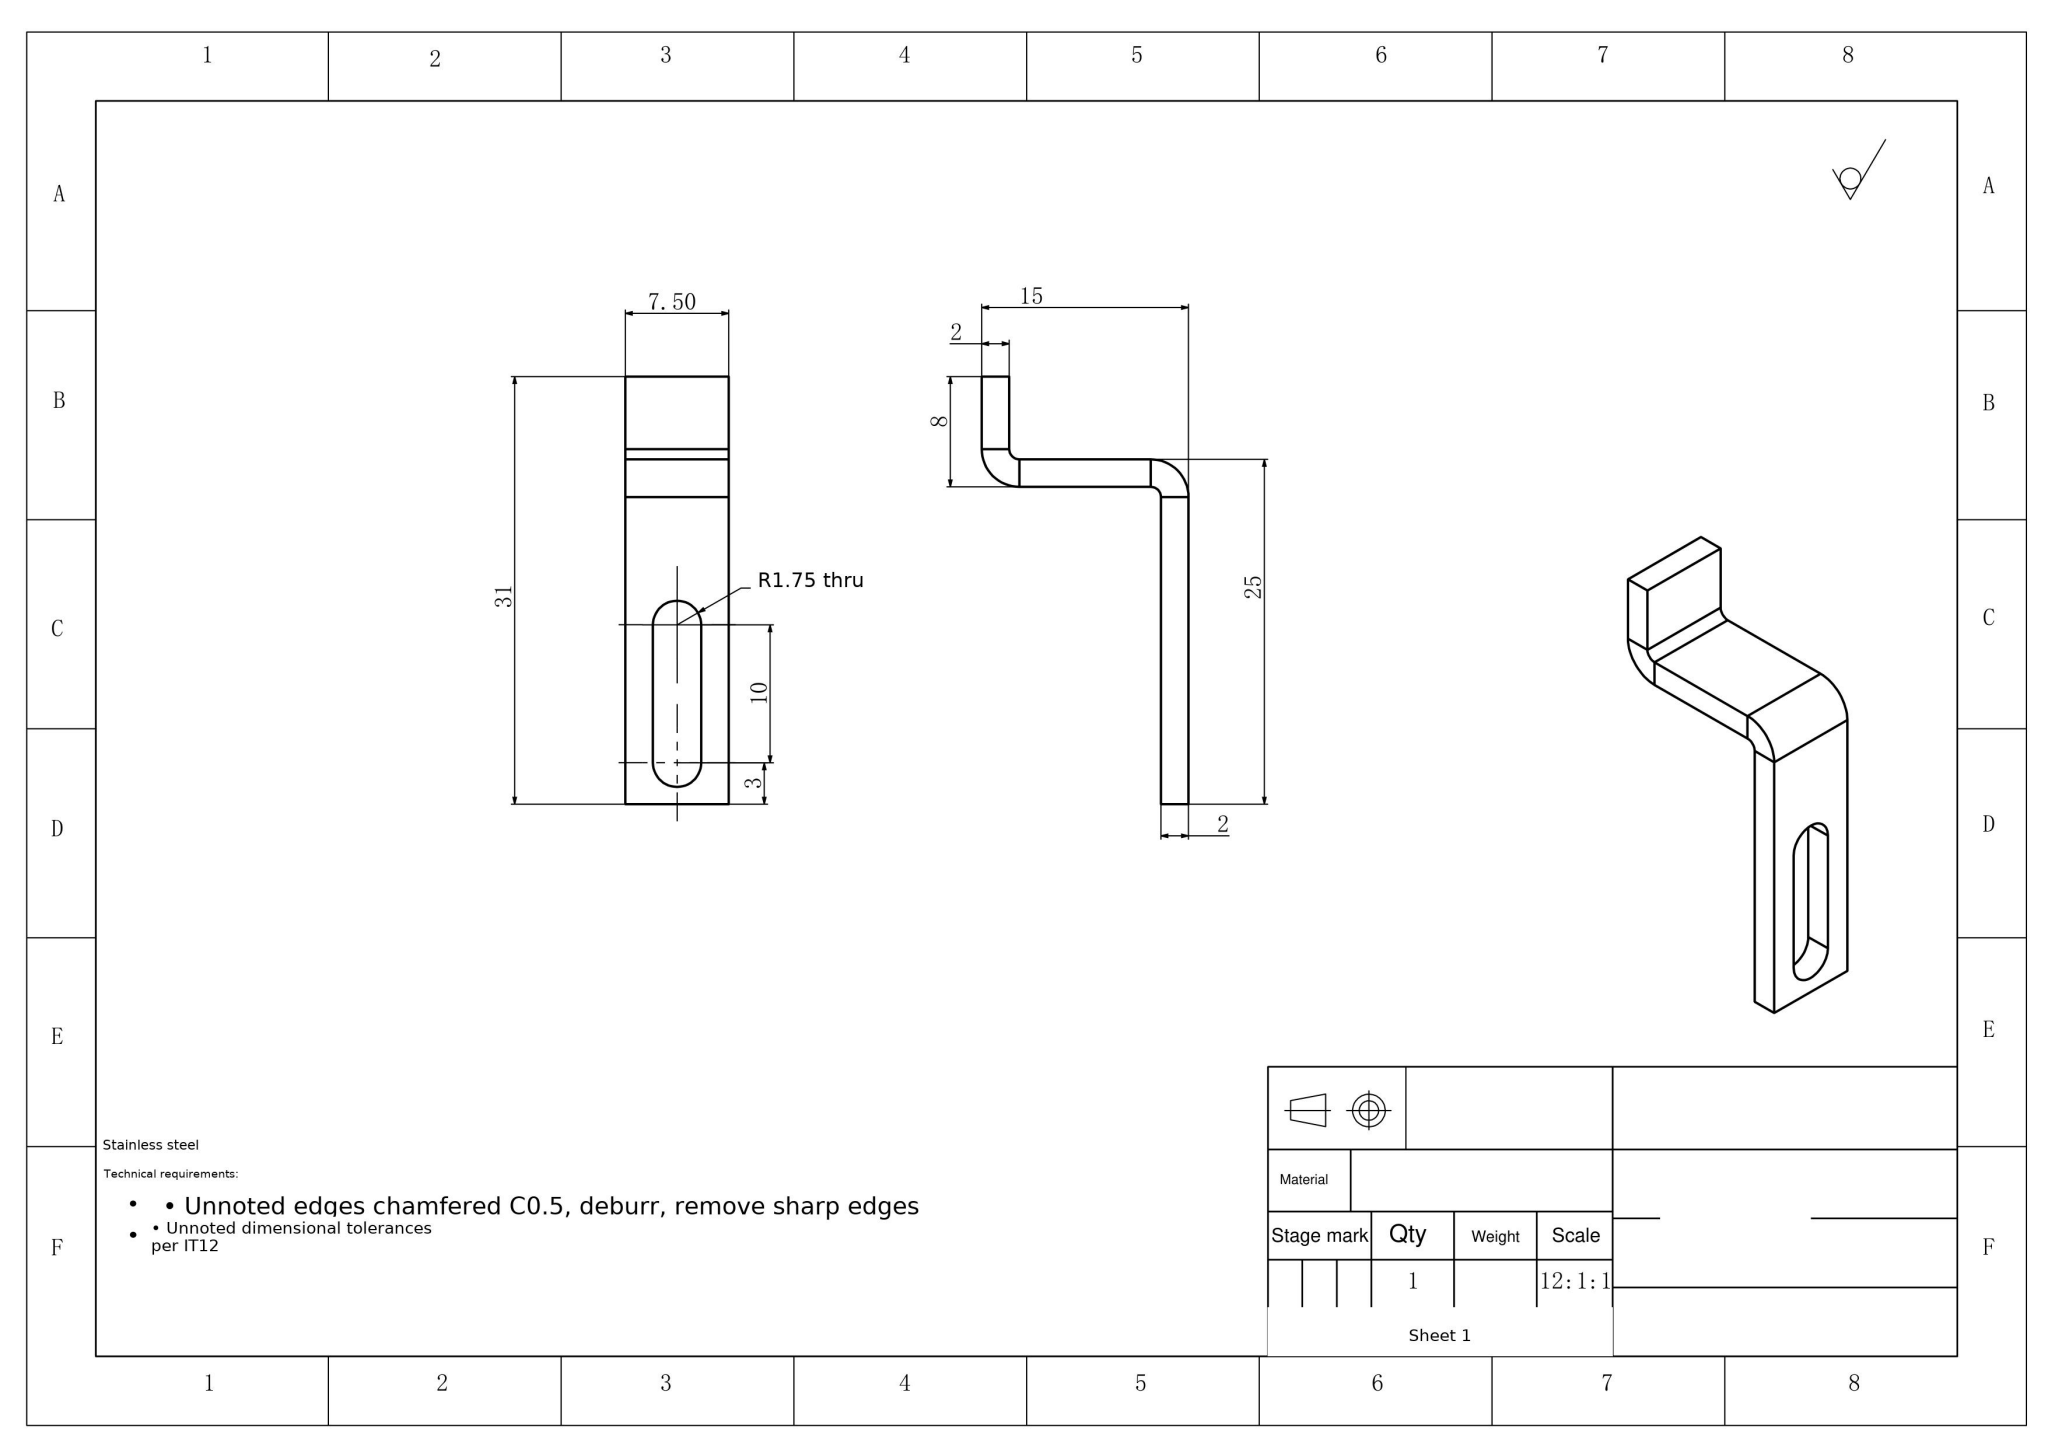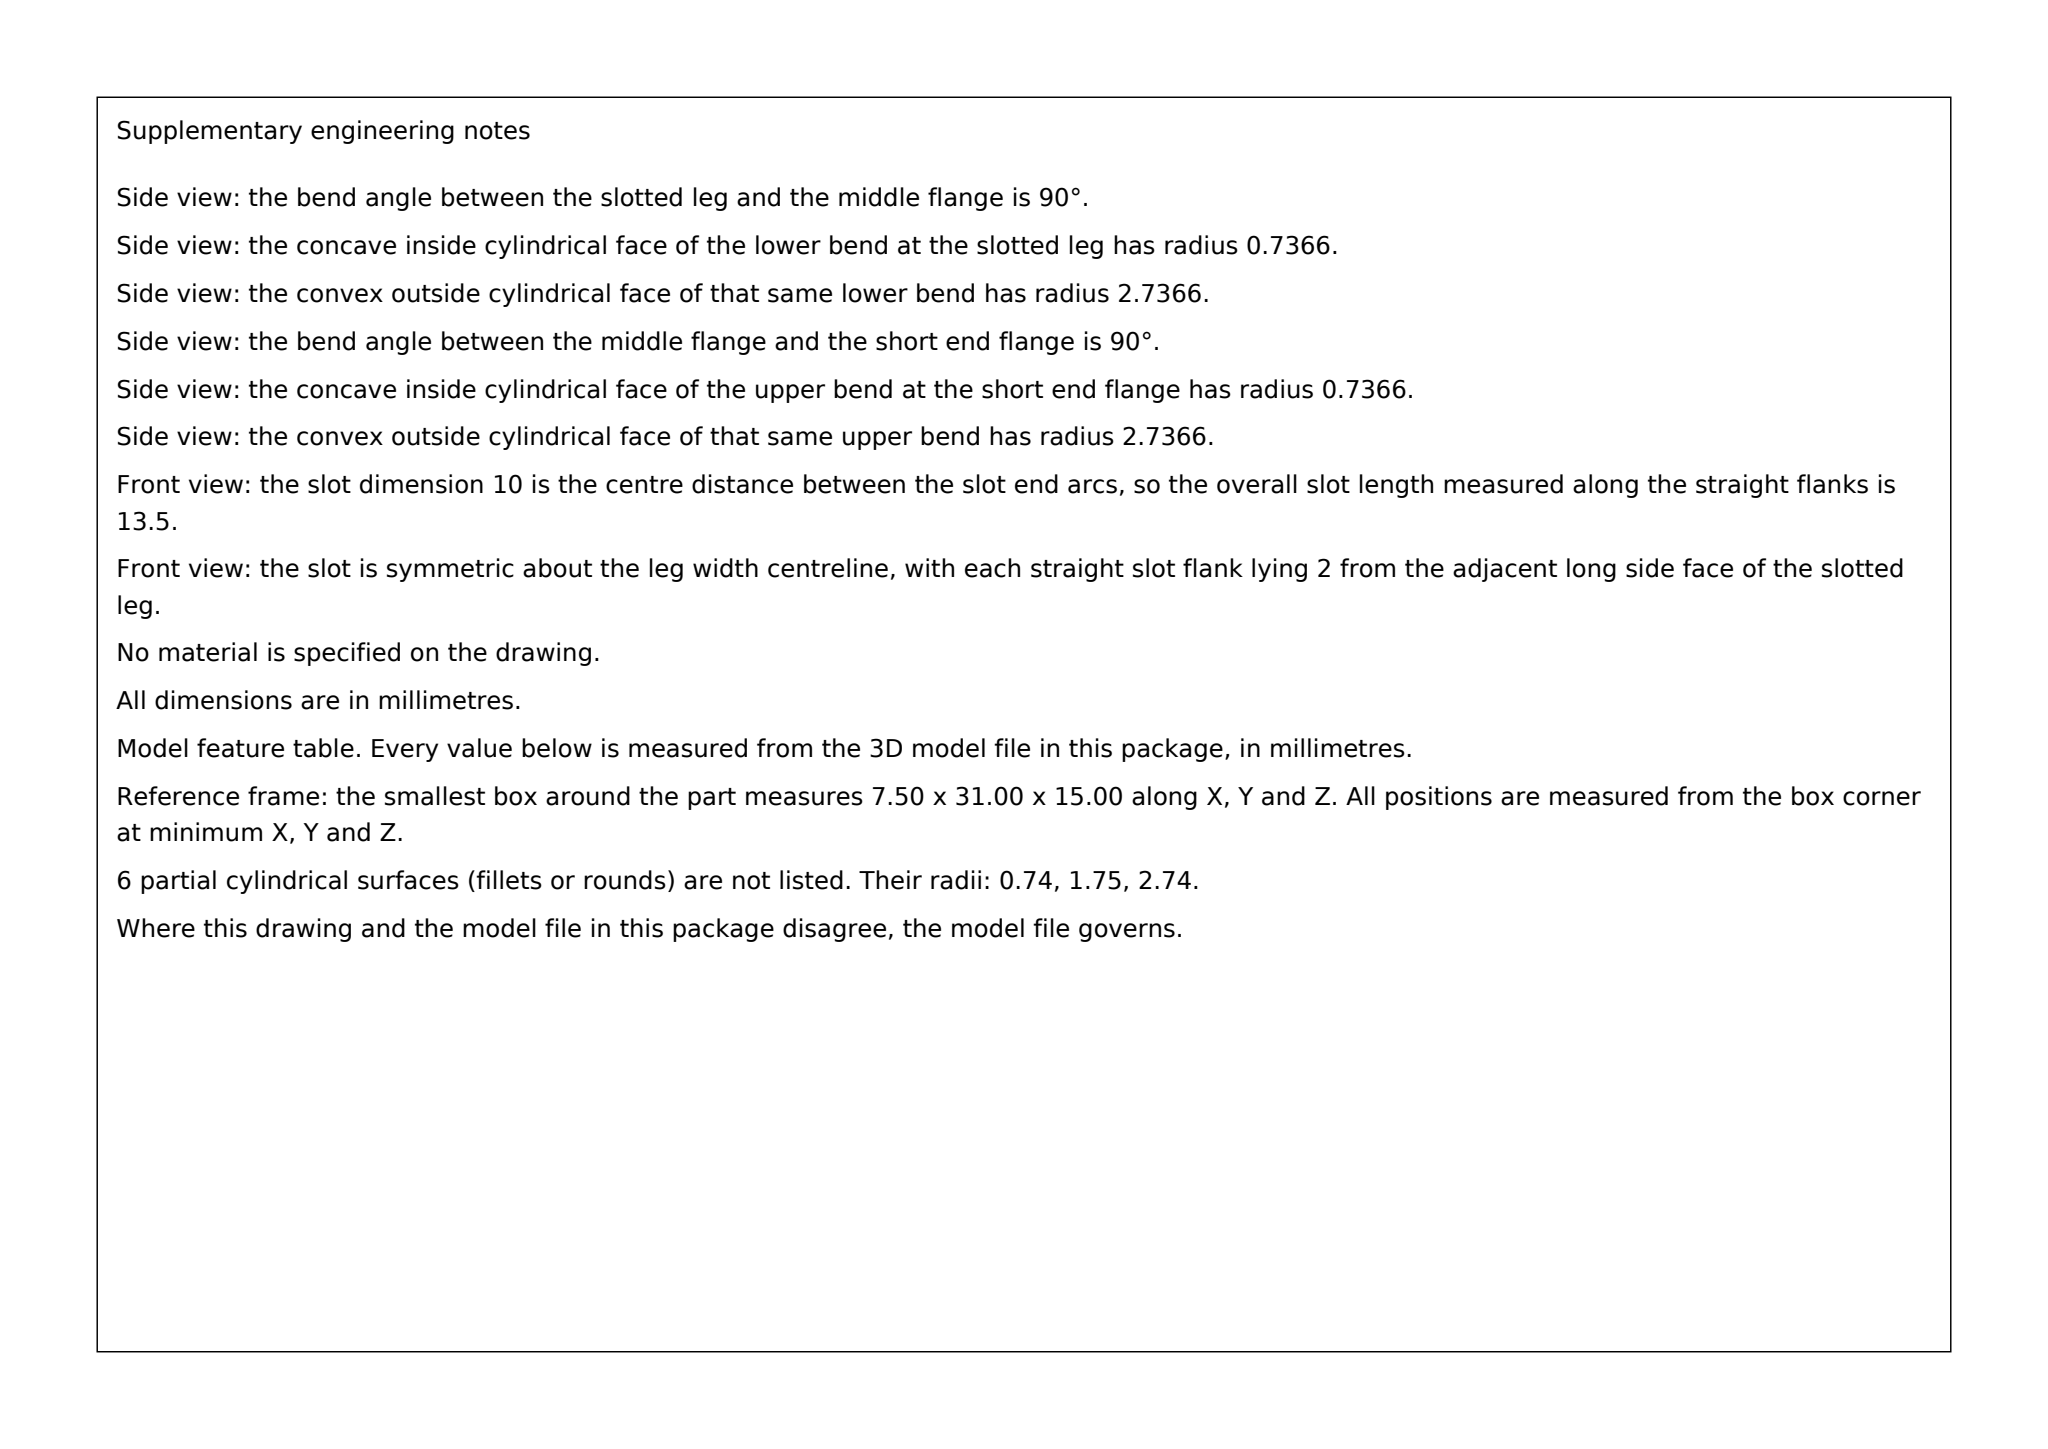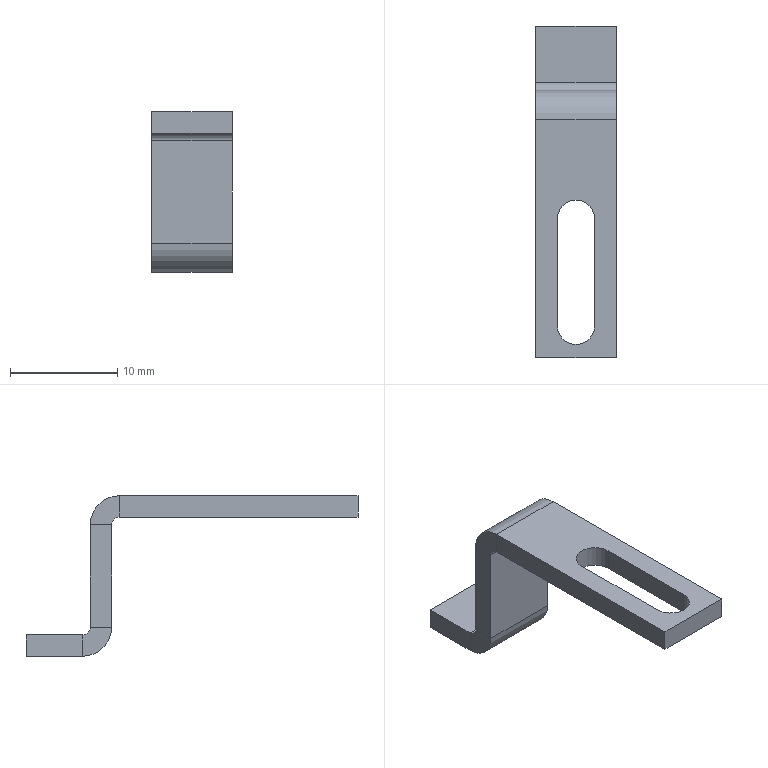Part | SolidWorks | mm | material Stainless steel | 1 solid | 26 faces | box 7.5 x 31 x 15 mm | volume 548 mm3 | plane 20 | cylinder 6 | commonest cylinder face diameters 3.5 x2 5.473 x2 1.473 x2
Drawing notes:
BEND FILLETS: 2X R0.74 INSIDE, 2X R2.74 OUTSIDE (DEL BALLOON 11) | from the solid: Cylinders dia 1.473 (R0.74) x2 and dia 5.473 (R2.74) x2, axis X, at y/z 22.26/12.26 and 25.74/2.74, length 7.5 = full width; inner/outer radii of the two 90 deg bends
STEP:
#1=CARTESIAN_POINT('',(3.75,12.5,-12.263));
#2=VERTEX_POINT('',#1);
#3=CARTESIAN_POINT('',(3.75,10.5,-12.263));
#4=VERTEX_POINT('',#3);
#5=CARTESIAN_POINT('',(3.75,12.5,-12.263));
#6=DIRECTION('',(0.,-1.,-0.));
#7=VECTOR('',#6,1000.);
#8=LINE('',#5,#7);
#9=EDGE_CURVE('',#2,#4,#8,.T.);
#10=ORIENTED_EDGE('',*,*,#9,.F.);
#11=CARTESIAN_POINT('',(3.75,12.5,-2.737));
#12=VERTEX_POINT('',#11);
#13=CARTESIAN_POINT('',(3.75,12.5,0.));
#14=DIRECTION('',(0.,0.,-1.));
#15=VECTOR('',#14,1000.);
#16=LINE('',#13,#15);
#17=EDGE_CURVE('',#12,#2,#16,.T.);
#18=ORIENTED_EDGE('',*,*,#17,.F.);
#19=CARTESIAN_POINT('',(3.75,10.5,-2.737));
#20=VERTEX_POINT('',#19);
#21=CARTESIAN_POINT('',(3.75,10.5,-2.737));
#22=DIRECTION('',(0.,1.,0.));
#23=VECTOR('',#22,1000.);
#24=LINE('',#21,#23);
#25=EDGE_CURVE('',#20,#12,#24,.T.);
#26=ORIENTED_EDGE('',*,*,#25,.F.);
#27=CARTESIAN_POINT('',(3.75,10.5,-15.));
#28=DIRECTION('',(0.,0.,-1.));
#29=VECTOR('',#28,1000.);
#30=LINE('',#27,#29);
#31=EDGE_CURVE('',#20,#4,#30,.T.);
#32=ORIENTED_EDGE('',*,*,#31,.T.);
#33=EDGE_LOOP('',(#10,#18,#26,#32));
#34=FACE_OUTER_BOUND('',#33,.T.);
#35=CARTESIAN_POINT('',(3.75,12.5,-15.));
#36=DIRECTION('',(-1.,0.,0.));
#37=DIRECTION('',(0.,0.,1.));
#38=AXIS2_PLACEMENT_3D('',#35,#36,#37);
#39=PLANE('',#38);
#40=ADVANCED_FACE('',(#34),#39,.F.);
#41=CARTESIAN_POINT('',(-3.75,12.5,-12.263));
#42=VERTEX_POINT('',#41);
#43=CARTESIAN_POINT('',(-3.75,10.5,-12.263));
#44=VERTEX_POINT('',#43);
#45=CARTESIAN_POINT('',(-3.75,12.5,-12.263));
#46=DIRECTION('',(-0.,-1.,-0.));
#47=VECTOR('',#46,1000.);
#48=LINE('',#45,#47);
#49=EDGE_CURVE('',#42,#44,#48,.T.);
#50=ORIENTED_EDGE('',*,*,#49,.T.);
#51=CARTESIAN_POINT('',(-3.75,10.5,-2.737));
#52=VERTEX_POINT('',#51);
#53=CARTESIAN_POINT('',(-3.75,10.5,-2.));
#54=DIRECTION('',(0.,-0.,1.));
#55=VECTOR('',#54,1000.);
#56=LINE('',#53,#55);
#57=EDGE_CURVE('',#44,#52,#56,.T.);
#58=ORIENTED_EDGE('',*,*,#57,.T.);
#59=CARTESIAN_POINT('',(-3.75,12.5,-2.737));
#60=VERTEX_POINT('',#59);
#61=CARTESIAN_POINT('',(-3.75,12.5,-2.737));
#62=DIRECTION('',(0.,1.,0.));
#63=VECTOR('',#62,1000.);
#64=LINE('',#61,#63);
#65=EDGE_CURVE('',#52,#60,#64,.T.);
#66=ORIENTED_EDGE('',*,*,#65,.T.);
#67=CARTESIAN_POINT('',(-3.75,12.5,0.));
#68=DIRECTION('',(0.,-0.,1.));
#69=VECTOR('',#68,1000.);
#70=LINE('',#67,#69);
#71=EDGE_CURVE('',#42,#60,#70,.T.);
#72=ORIENTED_EDGE('',*,*,#71,.F.);
#73=EDGE_LOOP('',(#50,#58,#66,#72));
#74=FACE_OUTER_BOUND('',#73,.T.);
#75=CARTESIAN_POINT('',(-3.75,12.5,-2.));
#76=DIRECTION('',(1.,0.,0.));
#77=DIRECTION('',(0.,0.,-1.));
#78=AXIS2_PLACEMENT_3D('',#75,#76,#77);
#79=PLANE('',#78);
#80=ADVANCED_FACE('',(#74),#79,.F.);
#81=CARTESIAN_POINT('',(-3.75,12.5,-12.263));
#82=DIRECTION('',(1.,0.,-0.));
#83=VECTOR('',#82,1000.);
#84=LINE('',#81,#83);
#85=EDGE_CURVE('',#42,#2,#84,.T.);
#86=ORIENTED_EDGE('',*,*,#85,.F.);
#87=ORIENTED_EDGE('',*,*,#71,.T.);
#88=CARTESIAN_POINT('',(-3.75,12.5,-2.737));
#89=DIRECTION('',(-1.,0.,0.));
#90=VECTOR('',#89,1000.);
#91=LINE('',#88,#90);
#92=EDGE_CURVE('',#12,#60,#91,.T.);
#93=ORIENTED_EDGE('',*,*,#92,.F.);
#94=ORIENTED_EDGE('',*,*,#17,.T.);
#95=EDGE_LOOP('',(#86,#87,#93,#94));
#96=FACE_OUTER_BOUND('',#95,.T.);
#97=CARTESIAN_POINT('',(0.,12.5,0.));
#98=DIRECTION('',(0.,-1.,-0.));
#99=DIRECTION('',(0.,0.,-1.));
#100=AXIS2_PLACEMENT_3D('',#97,#98,#99);
#101=PLANE('',#100);
#102=ADVANCED_FACE('',(#96),#101,.F.);
#103=ORIENTED_EDGE('',*,*,#57,.F.);
#104=CARTESIAN_POINT('',(-3.75,10.5,-12.263));
#105=DIRECTION('',(1.,0.,-0.));
#106=VECTOR('',#105,1000.);
#107=LINE('',#104,#106);
#108=EDGE_CURVE('',#44,#4,#107,.T.);
#109=ORIENTED_EDGE('',*,*,#108,.T.);
#110=ORIENTED_EDGE('',*,*,#31,.F.);
#111=CARTESIAN_POINT('',(-3.75,10.5,-2.737));
#112=DIRECTION('',(1.,0.,0.));
#113=VECTOR('',#112,1000.);
#114=LINE('',#111,#113);
#115=EDGE_CURVE('',#52,#20,#114,.T.);
#116=ORIENTED_EDGE('',*,*,#115,.F.);
#117=EDGE_LOOP('',(#103,#109,#110,#116));
#118=FACE_OUTER_BOUND('',#117,.T.);
#119=CARTESIAN_POINT('',(0.,10.5,0.));
#120=DIRECTION('',(0.,-1.,-0.));
#121=DIRECTION('',(0.,0.,-1.));
#122=AXIS2_PLACEMENT_3D('',#119,#120,#121);
#123=PLANE('',#122);
#124=ADVANCED_FACE('',(#118),#123,.T.);
#125=CARTESIAN_POINT('',(3.75,-12.5,-2.));
#126=VERTEX_POINT('',#125);
#127=CARTESIAN_POINT('',(3.75,9.763,-2.));
#128=VERTEX_POINT('',#127);
#129=CARTESIAN_POINT('',(3.75,-12.5,-2.));
#130=DIRECTION('',(0.,1.,0.));
#131=VECTOR('',#130,1000.);
#132=LINE('',#129,#131);
#133=EDGE_CURVE('',#126,#128,#132,.T.);
#134=ORIENTED_EDGE('',*,*,#133,.T.);
#135=CARTESIAN_POINT('',(3.75,9.763,0.));
#136=VERTEX_POINT('',#135);
#137=CARTESIAN_POINT('',(3.75,9.763,-2.));
#138=DIRECTION('',(0.,0.,1.));
#139=VECTOR('',#138,1000.);
#140=LINE('',#137,#139);
#141=EDGE_CURVE('',#128,#136,#140,.T.);
#142=ORIENTED_EDGE('',*,*,#141,.T.);
#143=CARTESIAN_POINT('',(3.75,-12.5,0.));
#144=VERTEX_POINT('',#143);
#145=CARTESIAN_POINT('',(3.75,-12.5,0.));
#146=DIRECTION('',(0.,1.,0.));
#147=VECTOR('',#146,1000.);
#148=LINE('',#145,#147);
#149=EDGE_CURVE('',#144,#136,#148,.T.);
#150=ORIENTED_EDGE('',*,*,#149,.F.);
#151=CARTESIAN_POINT('',(3.75,-12.5,-2.));
#152=DIRECTION('',(0.,0.,1.));
#153=VECTOR('',#152,1000.);
#154=LINE('',#151,#153);
#155=EDGE_CURVE('',#126,#144,#154,.T.);
#156=ORIENTED_EDGE('',*,*,#155,.F.);
#157=EDGE_LOOP('',(#134,#142,#150,#156));
#158=FACE_OUTER_BOUND('',#157,.T.);
#159=CARTESIAN_POINT('',(3.75,-12.5,-2.));
#160=DIRECTION('',(1.,0.,0.));
#161=DIRECTION('',(0.,0.,-1.));
#162=AXIS2_PLACEMENT_3D('',#159,#160,#161);
#163=PLANE('',#162);
#164=ADVANCED_FACE('',(#158),#163,.T.);
#165=CARTESIAN_POINT('',(1.75,0.5,-2.));
#166=VERTEX_POINT('',#165);
#167=CARTESIAN_POINT('',(-1.75,0.5,-2.));
#168=VERTEX_POINT('',#167);
#169=CARTESIAN_POINT('',(0.,0.5,-2.));
#170=DIRECTION('',(0.,0.,1.));
#171=DIRECTION('',(1.,0.,0.));
#172=AXIS2_PLACEMENT_3D('',#169,#170,#171);
#173=CIRCLE('',#172,1.75);
#174=EDGE_CURVE('',#166,#168,#173,.T.);
#175=ORIENTED_EDGE('',*,*,#174,.T.);
#176=CARTESIAN_POINT('',(-1.75,-9.5,-2.));
#177=VERTEX_POINT('',#176);
#178=CARTESIAN_POINT('',(-1.75,0.5,-2.));
#179=DIRECTION('',(0.,-1.,0.));
#180=VECTOR('',#179,1000.);
#181=LINE('',#178,#180);
#182=EDGE_CURVE('',#168,#177,#181,.T.);
#183=ORIENTED_EDGE('',*,*,#182,.T.);
#184=CARTESIAN_POINT('',(1.75,-9.5,-2.));
#185=VERTEX_POINT('',#184);
#186=CARTESIAN_POINT('',(0.,-9.5,-2.));
#187=DIRECTION('',(0.,0.,1.));
#188=DIRECTION('',(1.,0.,0.));
#189=AXIS2_PLACEMENT_3D('',#186,#187,#188);
#190=CIRCLE('',#189,1.75);
#191=EDGE_CURVE('',#177,#185,#190,.T.);
#192=ORIENTED_EDGE('',*,*,#191,.T.);
#193=CARTESIAN_POINT('',(1.75,0.5,-2.));
#194=DIRECTION('',(-0.,1.,0.));
#195=VECTOR('',#194,1000.);
#196=LINE('',#193,#195);
#197=EDGE_CURVE('',#185,#166,#196,.T.);
#198=ORIENTED_EDGE('',*,*,#197,.T.);
#199=EDGE_LOOP('',(#175,#183,#192,#198));
#200=FACE_BOUND('',#199,.T.);
#201=CARTESIAN_POINT('',(-3.75,9.763,-2.));
#202=VERTEX_POINT('',#201);
#203=CARTESIAN_POINT('',(-3.75,-12.5,-2.));
#204=VERTEX_POINT('',#203);
#205=CARTESIAN_POINT('',(-3.75,-12.5,-2.));
#206=DIRECTION('',(0.,-1.,0.));
#207=VECTOR('',#206,1000.);
#208=LINE('',#205,#207);
#209=EDGE_CURVE('',#202,#204,#208,.T.);
#210=ORIENTED_EDGE('',*,*,#209,.F.);
#211=CARTESIAN_POINT('',(3.75,9.763,-2.));
#212=DIRECTION('',(-1.,0.,0.));
#213=VECTOR('',#212,1000.);
#214=LINE('',#211,#213);
#215=EDGE_CURVE('',#128,#202,#214,.T.);
#216=ORIENTED_EDGE('',*,*,#215,.F.);
#217=ORIENTED_EDGE('',*,*,#133,.F.);
#218=CARTESIAN_POINT('',(-3.75,-12.5,-2.));
#219=DIRECTION('',(1.,0.,0.));
#220=VECTOR('',#219,1000.);
#221=LINE('',#218,#220);
#222=EDGE_CURVE('',#204,#126,#221,.T.);
#223=ORIENTED_EDGE('',*,*,#222,.F.);
#224=EDGE_LOOP('',(#210,#216,#217,#223));
#225=FACE_OUTER_BOUND('',#224,.T.);
#226=CARTESIAN_POINT('',(0.,0.,-2.));
#227=DIRECTION('',(0.,0.,-1.));
#228=DIRECTION('',(-1.,0.,0.));
#229=AXIS2_PLACEMENT_3D('',#226,#227,#228);
#230=PLANE('',#229);
#231=ADVANCED_FACE('',(#200,#225),#230,.T.);
#232=CARTESIAN_POINT('',(-1.75,0.5,0.));
#233=VERTEX_POINT('',#232);
#234=CARTESIAN_POINT('',(-1.75,-9.5,0.));
#235=VERTEX_POINT('',#234);
#236=CARTESIAN_POINT('',(-1.75,0.5,0.));
#237=DIRECTION('',(0.,-1.,0.));
#238=VECTOR('',#237,1000.);
#239=LINE('',#236,#238);
#240=EDGE_CURVE('',#233,#235,#239,.T.);
#241=ORIENTED_EDGE('',*,*,#240,.F.);
#242=CARTESIAN_POINT('',(1.75,0.5,0.));
#243=VERTEX_POINT('',#242);
#244=CARTESIAN_POINT('',(0.,0.5,0.));
#245=DIRECTION('',(0.,0.,1.));
#246=DIRECTION('',(1.,0.,0.));
#247=AXIS2_PLACEMENT_3D('',#244,#245,#246);
#248=CIRCLE('',#247,1.75);
#249=EDGE_CURVE('',#243,#233,#248,.T.);
#250=ORIENTED_EDGE('',*,*,#249,.F.);
#251=CARTESIAN_POINT('',(1.75,-9.5,0.));
#252=VERTEX_POINT('',#251);
#253=CARTESIAN_POINT('',(1.75,0.5,0.));
#254=DIRECTION('',(-0.,1.,0.));
#255=VECTOR('',#254,1000.);
#256=LINE('',#253,#255);
#257=EDGE_CURVE('',#252,#243,#256,.T.);
#258=ORIENTED_EDGE('',*,*,#257,.F.);
#259=CARTESIAN_POINT('',(0.,-9.5,0.));
#260=DIRECTION('',(0.,0.,1.));
#261=DIRECTION('',(1.,0.,0.));
#262=AXIS2_PLACEMENT_3D('',#259,#260,#261);
#263=CIRCLE('',#262,1.75);
#264=EDGE_CURVE('',#235,#252,#263,.T.);
#265=ORIENTED_EDGE('',*,*,#264,.F.);
#266=EDGE_LOOP('',(#241,#250,#258,#265));
#267=FACE_BOUND('',#266,.T.);
#268=CARTESIAN_POINT('',(-3.75,9.763,0.));
#269=VERTEX_POINT('',#268);
#270=CARTESIAN_POINT('',(3.75,9.763,0.));
#271=DIRECTION('',(-1.,0.,0.));
#272=VECTOR('',#271,1000.);
#273=LINE('',#270,#272);
#274=EDGE_CURVE('',#136,#269,#273,.T.);
#275=ORIENTED_EDGE('',*,*,#274,.T.);
#276=CARTESIAN_POINT('',(-3.75,-12.5,0.));
#277=VERTEX_POINT('',#276);
#278=CARTESIAN_POINT('',(-3.75,-12.5,0.));
#279=DIRECTION('',(0.,-1.,0.));
#280=VECTOR('',#279,1000.);
#281=LINE('',#278,#280);
#282=EDGE_CURVE('',#269,#277,#281,.T.);
#283=ORIENTED_EDGE('',*,*,#282,.T.);
#284=CARTESIAN_POINT('',(-3.75,-12.5,0.));
#285=DIRECTION('',(1.,0.,0.));
#286=VECTOR('',#285,1000.);
#287=LINE('',#284,#286);
#288=EDGE_CURVE('',#277,#144,#287,.T.);
#289=ORIENTED_EDGE('',*,*,#288,.T.);
#290=ORIENTED_EDGE('',*,*,#149,.T.);
#291=EDGE_LOOP('',(#275,#283,#289,#290));
#292=FACE_OUTER_BOUND('',#291,.T.);
#293=CARTESIAN_POINT('',(0.,0.,0.));
#294=DIRECTION('',(0.,0.,-1.));
#295=DIRECTION('',(-1.,0.,0.));
#296=AXIS2_PLACEMENT_3D('',#293,#294,#295);
#297=PLANE('',#296);
#298=ADVANCED_FACE('',(#267,#292),#297,.F.);
#299=ORIENTED_EDGE('',*,*,#288,.F.);
#300=CARTESIAN_POINT('',(-3.75,-12.5,-2.));
#301=DIRECTION('',(0.,0.,1.));
#302=VECTOR('',#301,1000.);
#303=LINE('',#300,#302);
#304=EDGE_CURVE('',#204,#277,#303,.T.);
#305=ORIENTED_EDGE('',*,*,#304,.F.);
#306=ORIENTED_EDGE('',*,*,#222,.T.);
#307=ORIENTED_EDGE('',*,*,#155,.T.);
#308=EDGE_LOOP('',(#299,#305,#306,#307));
#309=FACE_OUTER_BOUND('',#308,.T.);
#310=CARTESIAN_POINT('',(-3.75,-12.5,-2.));
#311=DIRECTION('',(0.,-1.,0.));
#312=DIRECTION('',(0.,0.,-1.));
#313=AXIS2_PLACEMENT_3D('',#310,#311,#312);
#314=PLANE('',#313);
#315=ADVANCED_FACE('',(#309),#314,.T.);
#316=CARTESIAN_POINT('',(-3.75,9.763,-2.));
#317=DIRECTION('',(0.,0.,1.));
#318=VECTOR('',#317,1000.);
#319=LINE('',#316,#318);
#320=EDGE_CURVE('',#202,#269,#319,.T.);
#321=ORIENTED_EDGE('',*,*,#320,.F.);
#322=ORIENTED_EDGE('',*,*,#209,.T.);
#323=ORIENTED_EDGE('',*,*,#304,.T.);
#324=ORIENTED_EDGE('',*,*,#282,.F.);
#325=EDGE_LOOP('',(#321,#322,#323,#324));
#326=FACE_OUTER_BOUND('',#325,.T.);
#327=CARTESIAN_POINT('',(-3.75,-12.5,-2.));
#328=DIRECTION('',(-1.,0.,0.));
#329=DIRECTION('',(0.,0.,1.));
#330=AXIS2_PLACEMENT_3D('',#327,#328,#329);
#331=PLANE('',#330);
#332=ADVANCED_FACE('',(#326),#331,.T.);
#333=ORIENTED_EDGE('',*,*,#249,.T.);
#334=CARTESIAN_POINT('',(-1.75,0.5,-2.));
#335=DIRECTION('',(0.,0.,1.));
#336=VECTOR('',#335,1000.);
#337=LINE('',#334,#336);
#338=EDGE_CURVE('',#168,#233,#337,.T.);
#339=ORIENTED_EDGE('',*,*,#338,.F.);
#340=ORIENTED_EDGE('',*,*,#174,.F.);
#341=CARTESIAN_POINT('',(1.75,0.5,-2.));
#342=DIRECTION('',(0.,0.,1.));
#343=VECTOR('',#342,1000.);
#344=LINE('',#341,#343);
#345=EDGE_CURVE('',#166,#243,#344,.T.);
#346=ORIENTED_EDGE('',*,*,#345,.T.);
#347=EDGE_LOOP('',(#333,#339,#340,#346));
#348=FACE_OUTER_BOUND('',#347,.T.);
#349=CARTESIAN_POINT('',(0.,0.5,-2.));
#350=DIRECTION('',(0.,0.,1.));
#351=DIRECTION('',(1.,0.,0.));
#352=AXIS2_PLACEMENT_3D('',#349,#350,#351);
#353=CYLINDRICAL_SURFACE('',#352,1.75);
#354=ADVANCED_FACE('',(#348),#353,.F.);
#355=ORIENTED_EDGE('',*,*,#257,.T.);
#356=ORIENTED_EDGE('',*,*,#345,.F.);
#357=ORIENTED_EDGE('',*,*,#197,.F.);
#358=CARTESIAN_POINT('',(1.75,-9.5,-2.));
#359=DIRECTION('',(0.,0.,1.));
#360=VECTOR('',#359,1000.);
#361=LINE('',#358,#360);
#362=EDGE_CURVE('',#185,#252,#361,.T.);
#363=ORIENTED_EDGE('',*,*,#362,.T.);
#364=EDGE_LOOP('',(#355,#356,#357,#363));
#365=FACE_OUTER_BOUND('',#364,.T.);
#366=CARTESIAN_POINT('',(1.75,0.5,-2.));
#367=DIRECTION('',(1.,0.,0.));
#368=DIRECTION('',(-0.,1.,0.));
#369=AXIS2_PLACEMENT_3D('',#366,#367,#368);
#370=PLANE('',#369);
#371=ADVANCED_FACE('',(#365),#370,.F.);
#372=ORIENTED_EDGE('',*,*,#264,.T.);
#373=ORIENTED_EDGE('',*,*,#362,.F.);
#374=ORIENTED_EDGE('',*,*,#191,.F.);
#375=CARTESIAN_POINT('',(-1.75,-9.5,-2.));
#376=DIRECTION('',(0.,0.,1.));
#377=VECTOR('',#376,1000.);
#378=LINE('',#375,#377);
#379=EDGE_CURVE('',#177,#235,#378,.T.);
#380=ORIENTED_EDGE('',*,*,#379,.T.);
#381=EDGE_LOOP('',(#372,#373,#374,#380));
#382=FACE_OUTER_BOUND('',#381,.T.);
#383=CARTESIAN_POINT('',(0.,-9.5,-2.));
#384=DIRECTION('',(0.,0.,1.));
#385=DIRECTION('',(1.,0.,0.));
#386=AXIS2_PLACEMENT_3D('',#383,#384,#385);
#387=CYLINDRICAL_SURFACE('',#386,1.75);
#388=ADVANCED_FACE('',(#382),#387,.F.);
#389=ORIENTED_EDGE('',*,*,#240,.T.);
#390=ORIENTED_EDGE('',*,*,#379,.F.);
#391=ORIENTED_EDGE('',*,*,#182,.F.);
#392=ORIENTED_EDGE('',*,*,#338,.T.);
#393=EDGE_LOOP('',(#389,#390,#391,#392));
#394=FACE_OUTER_BOUND('',#393,.T.);
#395=CARTESIAN_POINT('',(-1.75,0.5,-2.));
#396=DIRECTION('',(-1.,-0.,0.));
#397=DIRECTION('',(0.,-1.,0.));
#398=AXIS2_PLACEMENT_3D('',#395,#396,#397);
#399=PLANE('',#398);
#400=ADVANCED_FACE('',(#394),#399,.F.);
#401=ORIENTED_EDGE('',*,*,#65,.F.);
#402=CARTESIAN_POINT('',(-3.75,9.763,-2.737));
#403=DIRECTION('',(-1.,0.,0.));
#404=DIRECTION('',(0.,0.,-1.));
#405=AXIS2_PLACEMENT_3D('',#402,#403,#404);
#406=CIRCLE('',#405,0.7366);
#407=EDGE_CURVE('',#202,#52,#406,.T.);
#408=ORIENTED_EDGE('',*,*,#407,.F.);
#409=ORIENTED_EDGE('',*,*,#320,.T.);
#410=CARTESIAN_POINT('',(-3.75,9.763,-2.737));
#411=DIRECTION('',(-1.,0.,0.));
#412=DIRECTION('',(0.,0.,-1.));
#413=AXIS2_PLACEMENT_3D('',#410,#411,#412);
#414=CIRCLE('',#413,2.737);
#415=EDGE_CURVE('',#269,#60,#414,.T.);
#416=ORIENTED_EDGE('',*,*,#415,.T.);
#417=EDGE_LOOP('',(#401,#408,#409,#416));
#418=FACE_OUTER_BOUND('',#417,.T.);
#419=CARTESIAN_POINT('',(-3.75,9.763,-2.737));
#420=DIRECTION('',(-1.,0.,0.));
#421=DIRECTION('',(0.,0.,1.));
#422=AXIS2_PLACEMENT_3D('',#419,#420,#421);
#423=PLANE('',#422);
#424=ADVANCED_FACE('',(#418),#423,.T.);
#425=CARTESIAN_POINT('',(3.75,9.763,-2.737));
#426=DIRECTION('',(1.,0.,0.));
#427=DIRECTION('',(0.,0.,-1.));
#428=AXIS2_PLACEMENT_3D('',#425,#426,#427);
#429=CIRCLE('',#428,0.7366);
#430=EDGE_CURVE('',#20,#128,#429,.T.);
#431=ORIENTED_EDGE('',*,*,#430,.F.);
#432=ORIENTED_EDGE('',*,*,#25,.T.);
#433=CARTESIAN_POINT('',(3.75,9.763,-2.737));
#434=DIRECTION('',(1.,0.,0.));
#435=DIRECTION('',(0.,0.,-1.));
#436=AXIS2_PLACEMENT_3D('',#433,#434,#435);
#437=CIRCLE('',#436,2.737);
#438=EDGE_CURVE('',#12,#136,#437,.T.);
#439=ORIENTED_EDGE('',*,*,#438,.T.);
#440=ORIENTED_EDGE('',*,*,#141,.F.);
#441=EDGE_LOOP('',(#431,#432,#439,#440));
#442=FACE_OUTER_BOUND('',#441,.T.);
#443=CARTESIAN_POINT('',(3.75,9.763,-2.737));
#444=DIRECTION('',(-1.,0.,0.));
#445=DIRECTION('',(0.,0.,1.));
#446=AXIS2_PLACEMENT_3D('',#443,#444,#445);
#447=PLANE('',#446);
#448=ADVANCED_FACE('',(#442),#447,.F.);
#449=ORIENTED_EDGE('',*,*,#274,.F.);
#450=ORIENTED_EDGE('',*,*,#438,.F.);
#451=ORIENTED_EDGE('',*,*,#92,.T.);
#452=ORIENTED_EDGE('',*,*,#415,.F.);
#453=EDGE_LOOP('',(#449,#450,#451,#452));
#454=FACE_OUTER_BOUND('',#453,.T.);
#455=CARTESIAN_POINT('',(3.75,9.763,-2.737));
#456=DIRECTION('',(1.,0.,0.));
#457=DIRECTION('',(0.,1.,0.));
#458=AXIS2_PLACEMENT_3D('',#455,#456,#457);
#459=CYLINDRICAL_SURFACE('',#458,2.737);
#460=ADVANCED_FACE('',(#454),#459,.T.);
#461=ORIENTED_EDGE('',*,*,#215,.T.);
#462=ORIENTED_EDGE('',*,*,#407,.T.);
#463=ORIENTED_EDGE('',*,*,#115,.T.);
#464=ORIENTED_EDGE('',*,*,#430,.T.);
#465=EDGE_LOOP('',(#461,#462,#463,#464));
#466=FACE_OUTER_BOUND('',#465,.T.);
#467=CARTESIAN_POINT('',(3.75,9.763,-2.737));
#468=DIRECTION('',(1.,0.,0.));
#469=DIRECTION('',(0.,1.,0.));
#470=AXIS2_PLACEMENT_3D('',#467,#468,#469);
#471=CYLINDRICAL_SURFACE('',#470,0.7366);
#472=ADVANCED_FACE('',(#466),#471,.F.);
#473=CARTESIAN_POINT('',(3.75,13.237,-13.));
#474=VERTEX_POINT('',#473);
#475=CARTESIAN_POINT('',(3.75,13.237,-15.));
#476=VERTEX_POINT('',#475);
#477=CARTESIAN_POINT('',(3.75,13.237,-15.));
#478=DIRECTION('',(0.,0.,-1.));
#479=VECTOR('',#478,1000.);
#480=LINE('',#477,#479);
#481=EDGE_CURVE('',#474,#476,#480,.T.);
#482=ORIENTED_EDGE('',*,*,#481,.F.);
#483=CARTESIAN_POINT('',(3.75,13.237,-12.263));
#484=DIRECTION('',(1.,0.,-0.));
#485=DIRECTION('',(0.,0.,1.));
#486=AXIS2_PLACEMENT_3D('',#483,#484,#485);
#487=CIRCLE('',#486,0.7366);
#488=EDGE_CURVE('',#2,#474,#487,.T.);
#489=ORIENTED_EDGE('',*,*,#488,.F.);
#490=ORIENTED_EDGE('',*,*,#9,.T.);
#491=CARTESIAN_POINT('',(3.75,13.237,-12.263));
#492=DIRECTION('',(1.,0.,-0.));
#493=DIRECTION('',(0.,0.,1.));
#494=AXIS2_PLACEMENT_3D('',#491,#492,#493);
#495=CIRCLE('',#494,2.737);
#496=EDGE_CURVE('',#4,#476,#495,.T.);
#497=ORIENTED_EDGE('',*,*,#496,.T.);
#498=EDGE_LOOP('',(#482,#489,#490,#497));
#499=FACE_OUTER_BOUND('',#498,.T.);
#500=CARTESIAN_POINT('',(3.75,13.237,-12.263));
#501=DIRECTION('',(1.,0.,-0.));
#502=DIRECTION('',(-0.,0.,-1.));
#503=AXIS2_PLACEMENT_3D('',#500,#501,#502);
#504=PLANE('',#503);
#505=ADVANCED_FACE('',(#499),#504,.T.);
#506=CARTESIAN_POINT('',(-3.75,13.237,-13.));
#507=VERTEX_POINT('',#506);
#508=CARTESIAN_POINT('',(-3.75,13.237,-12.263));
#509=DIRECTION('',(-1.,0.,0.));
#510=DIRECTION('',(0.,0.,1.));
#511=AXIS2_PLACEMENT_3D('',#508,#509,#510);
#512=CIRCLE('',#511,0.7366);
#513=EDGE_CURVE('',#507,#42,#512,.T.);
#514=ORIENTED_EDGE('',*,*,#513,.F.);
#515=CARTESIAN_POINT('',(-3.75,13.237,-15.));
#516=VERTEX_POINT('',#515);
#517=CARTESIAN_POINT('',(-3.75,13.237,-13.));
#518=DIRECTION('',(0.,0.,-1.));
#519=VECTOR('',#518,1000.);
#520=LINE('',#517,#519);
#521=EDGE_CURVE('',#507,#516,#520,.T.);
#522=ORIENTED_EDGE('',*,*,#521,.T.);
#523=CARTESIAN_POINT('',(-3.75,13.237,-12.263));
#524=DIRECTION('',(-1.,0.,0.));
#525=DIRECTION('',(0.,0.,1.));
#526=AXIS2_PLACEMENT_3D('',#523,#524,#525);
#527=CIRCLE('',#526,2.737);
#528=EDGE_CURVE('',#516,#44,#527,.T.);
#529=ORIENTED_EDGE('',*,*,#528,.T.);
#530=ORIENTED_EDGE('',*,*,#49,.F.);
#531=EDGE_LOOP('',(#514,#522,#529,#530));
#532=FACE_OUTER_BOUND('',#531,.T.);
#533=CARTESIAN_POINT('',(-3.75,13.237,-12.263));
#534=DIRECTION('',(1.,0.,-0.));
#535=DIRECTION('',(-0.,0.,-1.));
#536=AXIS2_PLACEMENT_3D('',#533,#534,#535);
#537=PLANE('',#536);
#538=ADVANCED_FACE('',(#532),#537,.F.);
#539=ORIENTED_EDGE('',*,*,#108,.F.);
#540=ORIENTED_EDGE('',*,*,#528,.F.);
#541=CARTESIAN_POINT('',(3.75,13.237,-15.));
#542=DIRECTION('',(1.,0.,0.));
#543=VECTOR('',#542,1000.);
#544=LINE('',#541,#543);
#545=EDGE_CURVE('',#516,#476,#544,.T.);
#546=ORIENTED_EDGE('',*,*,#545,.T.);
#547=ORIENTED_EDGE('',*,*,#496,.F.);
#548=EDGE_LOOP('',(#539,#540,#546,#547));
#549=FACE_OUTER_BOUND('',#548,.T.);
#550=CARTESIAN_POINT('',(-3.75,13.237,-12.263));
#551=DIRECTION('',(-1.,0.,0.));
#552=DIRECTION('',(-0.,0.,-1.));
#553=AXIS2_PLACEMENT_3D('',#550,#551,#552);
#554=CYLINDRICAL_SURFACE('',#553,2.737);
#555=ADVANCED_FACE('',(#549),#554,.T.);
#556=ORIENTED_EDGE('',*,*,#85,.T.);
#557=ORIENTED_EDGE('',*,*,#488,.T.);
#558=CARTESIAN_POINT('',(3.75,13.237,-13.));
#559=DIRECTION('',(-1.,0.,0.));
#560=VECTOR('',#559,1000.);
#561=LINE('',#558,#560);
#562=EDGE_CURVE('',#474,#507,#561,.T.);
#563=ORIENTED_EDGE('',*,*,#562,.T.);
#564=ORIENTED_EDGE('',*,*,#513,.T.);
#565=EDGE_LOOP('',(#556,#557,#563,#564));
#566=FACE_OUTER_BOUND('',#565,.T.);
#567=CARTESIAN_POINT('',(-3.75,13.237,-12.263));
#568=DIRECTION('',(-1.,0.,0.));
#569=DIRECTION('',(-0.,0.,-1.));
#570=AXIS2_PLACEMENT_3D('',#567,#568,#569);
#571=CYLINDRICAL_SURFACE('',#570,0.7366);
#572=ADVANCED_FACE('',(#566),#571,.F.);
#573=ORIENTED_EDGE('',*,*,#481,.T.);
#574=CARTESIAN_POINT('',(3.75,18.5,-15.));
#575=VERTEX_POINT('',#574);
#576=CARTESIAN_POINT('',(3.75,-0.,-15.));
#577=DIRECTION('',(0.,-1.,0.));
#578=VECTOR('',#577,1000.);
#579=LINE('',#576,#578);
#580=EDGE_CURVE('',#575,#476,#579,.T.);
#581=ORIENTED_EDGE('',*,*,#580,.F.);
#582=CARTESIAN_POINT('',(3.75,18.5,-13.));
#583=VERTEX_POINT('',#582);
#584=CARTESIAN_POINT('',(3.75,18.5,-15.));
#585=DIRECTION('',(0.,0.,1.));
#586=VECTOR('',#585,1000.);
#587=LINE('',#584,#586);
#588=EDGE_CURVE('',#575,#583,#587,.T.);
#589=ORIENTED_EDGE('',*,*,#588,.T.);
#590=CARTESIAN_POINT('',(3.75,12.5,-13.));
#591=DIRECTION('',(0.,-1.,0.));
#592=VECTOR('',#591,1000.);
#593=LINE('',#590,#592);
#594=EDGE_CURVE('',#583,#474,#593,.T.);
#595=ORIENTED_EDGE('',*,*,#594,.T.);
#596=EDGE_LOOP('',(#573,#581,#589,#595));
#597=FACE_OUTER_BOUND('',#596,.T.);
#598=CARTESIAN_POINT('',(3.75,12.5,-15.));
#599=DIRECTION('',(-1.,0.,0.));
#600=DIRECTION('',(0.,0.,1.));
#601=AXIS2_PLACEMENT_3D('',#598,#599,#600);
#602=PLANE('',#601);
#603=ADVANCED_FACE('',(#597),#602,.F.);
#604=ORIENTED_EDGE('',*,*,#521,.F.);
#605=CARTESIAN_POINT('',(-3.75,18.5,-13.));
#606=VERTEX_POINT('',#605);
#607=CARTESIAN_POINT('',(-3.75,18.5,-13.));
#608=DIRECTION('',(0.,1.,0.));
#609=VECTOR('',#608,1000.);
#610=LINE('',#607,#609);
#611=EDGE_CURVE('',#507,#606,#610,.T.);
#612=ORIENTED_EDGE('',*,*,#611,.T.);
#613=CARTESIAN_POINT('',(-3.75,18.5,-15.));
#614=VERTEX_POINT('',#613);
#615=CARTESIAN_POINT('',(-3.75,18.5,-15.));
#616=DIRECTION('',(0.,0.,1.));
#617=VECTOR('',#616,1000.);
#618=LINE('',#615,#617);
#619=EDGE_CURVE('',#614,#606,#618,.T.);
#620=ORIENTED_EDGE('',*,*,#619,.F.);
#621=CARTESIAN_POINT('',(-3.75,-0.,-15.));
#622=DIRECTION('',(0.,1.,0.));
#623=VECTOR('',#622,1000.);
#624=LINE('',#621,#623);
#625=EDGE_CURVE('',#516,#614,#624,.T.);
#626=ORIENTED_EDGE('',*,*,#625,.F.);
#627=EDGE_LOOP('',(#604,#612,#620,#626));
#628=FACE_OUTER_BOUND('',#627,.T.);
#629=CARTESIAN_POINT('',(-3.75,18.5,-15.));
#630=DIRECTION('',(1.,0.,0.));
#631=DIRECTION('',(0.,0.,-1.));
#632=AXIS2_PLACEMENT_3D('',#629,#630,#631);
#633=PLANE('',#632);
#634=ADVANCED_FACE('',(#628),#633,.F.);
#635=ORIENTED_EDGE('',*,*,#545,.F.);
#636=ORIENTED_EDGE('',*,*,#625,.T.);
#637=CARTESIAN_POINT('',(0.,18.5,-15.));
#638=DIRECTION('',(1.,0.,0.));
#639=VECTOR('',#638,1000.);
#640=LINE('',#637,#639);
#641=EDGE_CURVE('',#614,#575,#640,.T.);
#642=ORIENTED_EDGE('',*,*,#641,.T.);
#643=ORIENTED_EDGE('',*,*,#580,.T.);
#644=EDGE_LOOP('',(#635,#636,#642,#643));
#645=FACE_OUTER_BOUND('',#644,.T.);
#646=CARTESIAN_POINT('',(0.,-0.,-15.));
#647=DIRECTION('',(0.,0.,1.));
#648=DIRECTION('',(1.,0.,0.));
#649=AXIS2_PLACEMENT_3D('',#646,#647,#648);
#650=PLANE('',#649);
#651=ADVANCED_FACE('',(#645),#650,.F.);
#652=ORIENTED_EDGE('',*,*,#611,.F.);
#653=ORIENTED_EDGE('',*,*,#562,.F.);
#654=ORIENTED_EDGE('',*,*,#594,.F.);
#655=CARTESIAN_POINT('',(3.75,18.5,-13.));
#656=DIRECTION('',(1.,0.,0.));
#657=VECTOR('',#656,1000.);
#658=LINE('',#655,#657);
#659=EDGE_CURVE('',#606,#583,#658,.T.);
#660=ORIENTED_EDGE('',*,*,#659,.F.);
#661=EDGE_LOOP('',(#652,#653,#654,#660));
#662=FACE_OUTER_BOUND('',#661,.T.);
#663=CARTESIAN_POINT('',(0.,-0.,-13.));
#664=DIRECTION('',(0.,0.,1.));
#665=DIRECTION('',(1.,0.,0.));
#666=AXIS2_PLACEMENT_3D('',#663,#664,#665);
#667=PLANE('',#666);
#668=ADVANCED_FACE('',(#662),#667,.T.);
#669=ORIENTED_EDGE('',*,*,#659,.T.);
#670=ORIENTED_EDGE('',*,*,#588,.F.);
#671=ORIENTED_EDGE('',*,*,#641,.F.);
#672=ORIENTED_EDGE('',*,*,#619,.T.);
#673=EDGE_LOOP('',(#669,#670,#671,#672));
#674=FACE_OUTER_BOUND('',#673,.T.);
#675=CARTESIAN_POINT('',(3.75,18.5,-15.));
#676=DIRECTION('',(0.,-1.,0.));
#677=DIRECTION('',(0.,-0.,-1.));
#678=AXIS2_PLACEMENT_3D('',#675,#676,#677);
#679=PLANE('',#678);
#680=ADVANCED_FACE('',(#674),#679,.F.);
#681=CLOSED_SHELL('',(#40,#80,#102,#124,#164,#231,#298,#315,#332,#354,#371,#388,#400,#424,#448,#460,#472,#505,#538,#555,#572,#603,#634,#651,#668,#680));
#682=MANIFOLD_SOLID_BREP('',#681);
#683=CARTESIAN_POINT('',(0.,0.,0.));
#684=DIRECTION('',(0.,0.,1.));
#685=DIRECTION('',(1.,0.,0.));
#686=AXIS2_PLACEMENT_3D('',#683,#684,#685);
#687=(LENGTH_UNIT()NAMED_UNIT(*)SI_UNIT(.MILLI.,.METRE.));
#688=UNCERTAINTY_MEASURE_WITH_UNIT(LENGTH_MEASURE(0.00001),#687,'','');
#689=(NAMED_UNIT(*)PLANE_ANGLE_UNIT()SI_UNIT($,.RADIAN.));
#690=(NAMED_UNIT(*)SI_UNIT($,.STERADIAN.)SOLID_ANGLE_UNIT());
#691=(GEOMETRIC_REPRESENTATION_CONTEXT(3)GLOBAL_UNCERTAINTY_ASSIGNED_CONTEXT((#688))GLOBAL_UNIT_ASSIGNED_CONTEXT((#687,#689,#690))REPRESENTATION_CONTEXT('',''));
#692=ADVANCED_BREP_SHAPE_REPRESENTATION('',(#682,#686),#691);